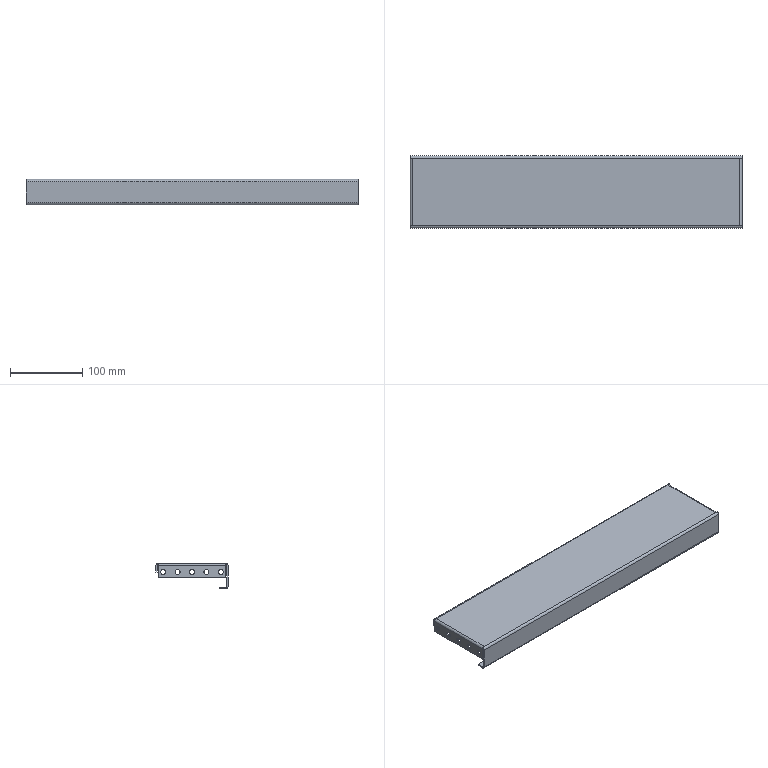Component | SolidWorks | UpperSeatAssembly-1_UpperSill-1 | 1 solid | 70 faces | volume 144110 mm3 | plane 40 | cylinder 30 | commonest cylinder face diameters 6.8 x20 6 x5 2 x5